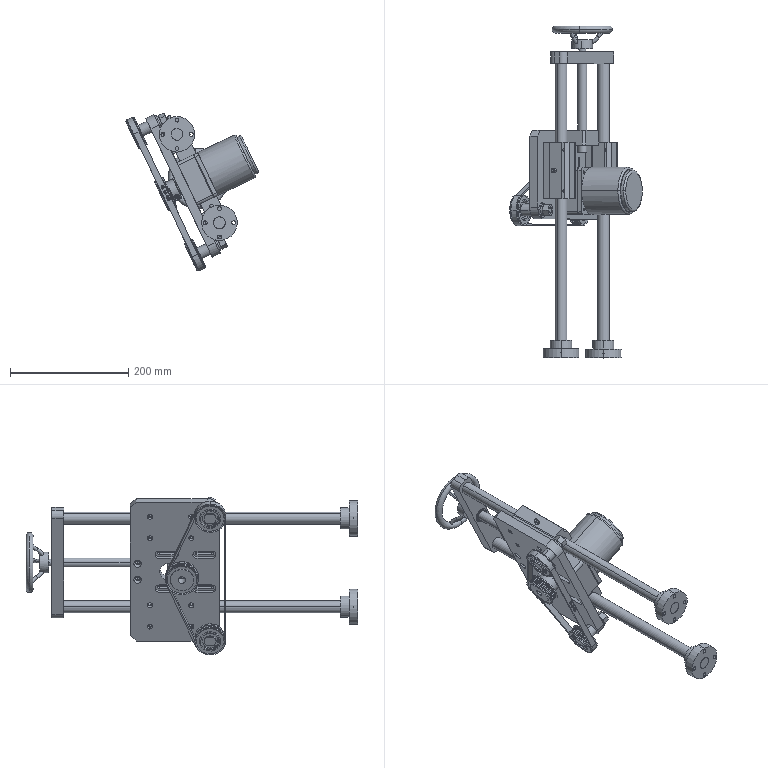Assembly | SolidWorks | mm | 32 component files | 32 solids | 1935 faces | box 224.34 x 561.5 x 267.03 mm | volume 2250519 mm3 | cylinder 1205 | plane 397 | cone 122 | torus 104 | spline 73 | sphere 34 | commonest cylinder face diameters 1.1 x224 0.5 x212 6.55 x196 46.79 x62 43.25 x60 46.43 x33 20 x32 49.97 x32
Bill of materials:
20OpticalAxis1-1 | 2 |  | Long, slender solid cylindrical rod with a constant diameter and plain flat ends.
25WMotor | 1 |  | Motor-like body: a cylindrical housing with a stepped, rounded rear end cap, joined to a square flange and a rectangular front block that has an output shaft sticking out of it.
AHTF30S5M100body | 2 |  | Toothed pulley-like ring: a short cylinder with axial teeth around its outside, a flange at each end, and a large central bore.
bearingB6201ZZ | 2 |  | Short annular ring with flat faces, a central bore, and concentric circular lines on the faces, looking like a simplified bearing.
RTWN32 | 2 |  | Thin, flat, open circular ring of constant thickness, with a lug at each end of the gap and a small hole through each lug, shaped like an internal retaining ring.
Bearing | 2 |  | Rectangular block housing with a large axial through-bore, stepped/chamfered side faces, mounting holes on the top and side faces, and a small fitting on the top, looking like a linear bushing block.
Rolling bearings 61901 GB 276-94 | 1 |  | Annular rolling-element assembly shaped like a radial ball bearing: concentric outer and inner rings with one ring of spherical balls between them, open on the visible face.
DowelPin1-1 | 2 |  | Headed stepped pin: a round head flange, a long cylindrical shank, and a shorter, smaller-diameter end, with a small ring/groove at the step.
FeedingOpticalAxisFrameConnector1-1 | 1 |  | Flat bar link with rounded ends: two small holes near the ends and a larger hole in the middle, with counterbores or chamfers on one face.
FeedingPressingPlate1-1 | 1 |  | Rectangular flat plate with one rounded and one chamfered corner, a central obround slot, four parallel slots, and many through-holes of several sizes in symmetric patterns.
FeedingPressingPlateAdjustmentBlock1-1 | 1 |  | Rectangular block with chamfers on two opposite edges and a single round through-hole crossing it.
FeedingPressingScrew1-1 | 1 |  | Solid stepped cylindrical shaft: a long main diameter that steps down twice to smaller diameters at one end.
Handle1-1 | 1 |  | Handwheel-like part: a toroidal rim joined by three curved spokes to a cylindrical hub that sits off the rim's plane and has a small central bore.
GB_FASTENER_NUT_SNAB1XY M12X1.5-N | 2 |  | Hexagonal prism with a central through-bore, shaped like a hex nut, with chamfered corners on both end faces.
HTCPA32_S5M100_12pulley | 1 |  | Toothed pulley: a cylindrical body with axial teeth around its outside, a flange on each side of the toothed section, and a cylindrical hub on one side. The hub has a central bore and a radial slit, which looks like a clamping hub.
Slotted_head_cap_screw_ISO_4762_M4x16 | 1 |  | Headed fastener: a cylindrical head with a hexagonal socket recess, a plain straight cylindrical shank, and a chamfered tip. The shape matches a socket-head cap screw.
OpticalAxisSeat1-1 | 2 |  | Flanged bushing or flange nut body: a round flange with a smaller cylindrical boss on one side, a central through bore, and four evenly spaced through holes on a bolt circle in the flange.
GB_FASTENER_WASHER_PWNA 12 | 2 |  | Thin, flat, plain annular disc with a central circular hole, shaped like a flat washer.
GB_FASTENER_WASHER_SW 12 | 2 |  | Ring with a rectangular cross-section and one radial split through the ring, shaped like a split (spring) lock washer.
TimingBelt5M-10-625 | 1 |  | Thin closed-loop band of constant width and thickness, shaped like a rounded triangle: one long straight side and two shorter sides meeting at rounded corners.
Washer1-1 | 2 |  | Plain cylindrical tube: a hollow cylinder with a concentric through bore and flat, square-cut ends, shaped like a spacer or sleeve.
Mates:
1. coincident | 20OpticalAxis1-1-1 face at (-30.965, 0, 663.073) dir (0, -1, 0) | assembly plane at (0, 0, 0) dir (0, 1, 0)
2. concentric | 20OpticalAxis1-1-1 face at (-30.965, 0, 663.073) dir (0, 1, 0) r 10 | Bearing-2 face at (-30.965, 269, 663.073) dir (0, -1, 0) r 10
3. concentric | 20OpticalAxis1-1-2 face at (40.711, 0, 513.345) dir (0, 1, 0) r 10 | Bearing-1 face at (40.711, 269, 513.345) dir (0, -1, 0) r 10
4. coincident | 20OpticalAxis1-1-1 face at (-30.965, 0, 663.073) dir (0, -1, 0) | 20OpticalAxis1-1-2 face at (40.711, 0, 513.345) dir (0, -1, 0)
5. coincident | Bearing-1 face at (33.428, 365, 479.924) dir (-0.902, 0, -0.4318) | Bearing-2 face at (-38.248, 365, 629.652) dir (-0.902, 0, -0.4318)
6. coincident | Bearing-1 face at (70.409, 365, 497.627) dir (0, 1, 0) | Bearing-2 face at (-1.267, 365, 647.355) dir (0, 1, 0)
7. concentric | 20OpticalAxis1-1-1 face at (-30.965, 0, 663.073) dir (0, 1, 0) r 10 | OpticalAxisSeat1-1-1 face at (-30.965, -1.22, 663.073) dir (0, -1, 0) r 10
8. coincident | 20OpticalAxis1-1-1 face at (-30.965, 0, 663.073) dir (0, -1, 0) | OpticalAxisSeat1-1-1 face at (-20.965, 0, 663.073) dir (0, -1, 0)
9. concentric | 20OpticalAxis1-1-2 face at (40.711, 0, 513.345) dir (0, 1, 0) r 10 | OpticalAxisSeat1-1-2 face at (40.711, -1.22, 513.345) dir (0, -1, 0) r 10
10. coincident | 20OpticalAxis1-1-2 face at (40.711, 0, 513.345) dir (0, -1, 0) | OpticalAxisSeat1-1-2 face at (50.711, 0, 513.345) dir (0, -1, 0)
11. coincident | Bearing-1 face at (33.428, 365, 479.924) dir (-0.902, 0, -0.4318) | FeedingPressingPlate1-1-1 face at (-70.2, 235, 696.399) dir (0.902, 0, 0.4318)
12. distance | Bearing-1 face at (70.409, 365, 497.627) dir (0, 1, 0) | FeedingPressingPlate1-1-1 face at (-70.2, 385, 696.399) dir (0, 1, 0)
13. distance | Bearing-2 face at (-107.114, 439.5, 656.554) dir (-0.4318, 0, 0.902) | FeedingPressingPlate1-1-1 face at (-70.2, 235, 696.399) dir (-0.4318, 0, 0.902)
14. concentric | FeedingPressingPlate1-1-1 face at (35.587, 250, 475.414) dir (-0.902, 0, -0.4318) r 6 | AHTF30S5M100-1/bearingB6201ZZ-1 face at (-5.002, 250, 455.984) dir (0.902, 0, 0.4318) r 6
15. concentric | FeedingPressingPlate1-1-1 face at (-63.723, 250, 682.869) dir (-0.902, 0, -0.4318) r 6 | AHTF30S5M100-2/bearingB6201ZZ-1 face at (-104.312, 250, 663.439) dir (0.902, 0, 0.4318) r 6
16. coincident | AHTF30S5M100-1/AHTF30S5M100body-1 face at (-10.355, 264.779, 460.218) dir (-0.902, 0, -0.4318) | AHTF30S5M100-2/AHTF30S5M100body-1 face at (-109.665, 264.779, 667.673) dir (-0.902, 0, -0.4318)
17. concentric | AHTF30S5M100-1/bearingB6201ZZ-1 face at (-5.002, 250, 455.984) dir (0.902, 0, 0.4318) r 6 | DowelPin1-1-1 face at (33.783, 250, 474.551) dir (-0.902, 0, -0.4318) r 6
18. coincident | AHTF30S5M100-1/bearingB6201ZZ-1 face at (-6.094, 256.096, 458.265) dir (-0.902, 0, -0.4318) | DowelPin1-1-1 face at (-5.002, 250, 455.984) dir (0.902, 0, 0.4318)
19. concentric | DowelPin1-1-1 face at (33.783, 250, 474.551) dir (-0.902, 0, -0.4318) r 6 | Washer1-1-1 face at (22.057, 250, 468.937) dir (-0.902, 0, -0.4318) r 6.25
20. coincident | AHTF30S5M100-1/bearingB6201ZZ-1 face at (2.578, 258.036, 463.308) dir (0.902, 0, 0.4318) | Washer1-1-1 face at (4.018, 250, 460.302) dir (-0.902, 0, -0.4318)
21. coincident | FeedingPressingPlate1-1-1 face at (-83.73, 235, 689.922) dir (-0.902, 0, -0.4318) | Washer1-1-1 face at (22.057, 250, 468.937) dir (0.902, 0, 0.4318)
22. concentric | DowelPin1-1-1 face at (49.116, 250, 481.891) dir (-0.902, 0, -0.4318) r 5.188 | hex nuts 1-fine pitch-grades ab gb-1 face at (40.638, 250, 477.832) dir (0.902, 0, 0.4318) r 523.599
23. coincident | hex nuts 1-fine pitch-grades ab gb-1 face at (38.394, 241, 482.519) dir (-0.902, 0, -0.4318) | spring lock washers--normal type gb-1 face at (40.638, 250, 477.832) dir (0.902, 0, 0.4318)
24. concentric | DowelPin1-1-1 face at (49.116, 250, 481.891) dir (-0.902, 0, -0.4318) r 5.188 | plain washers-n series-grade a gb-1 face at (37.842, 250, 476.494) dir (-0.902, 0, -0.4318) r 6.5
25. concentric | plain washers-n series-grade a gb-1 face at (37.842, 250, 476.494) dir (-0.902, 0, -0.4318) r 12 | spring lock washers--normal type gb-1 face at (37.842, 250, 476.494) dir (0.902, 0, 0.4318) r 6.45
26. coincident | plain washers-n series-grade a gb-1 face at (37.842, 250, 476.494) dir (0.902, 0, 0.4318) | spring lock washers--normal type gb-1 face at (37.842, 250, 476.494) dir (-0.902, 0, -0.4318)
27. coincident | FeedingPressingPlate1-1-1 face at (-70.2, 235, 696.399) dir (0.902, 0, 0.4318) | plain washers-n series-grade a gb-1 face at (35.587, 250, 475.414) dir (-0.902, 0, -0.4318)
28. concentric | AHTF30S5M100-2/bearingB6201ZZ-1 face at (-104.312, 250, 663.439) dir (0.902, 0, 0.4318) r 6 | DowelPin1-1-2 face at (-65.527, 250, 682.005) dir (-0.902, 0, -0.4318) r 6
29. coincident | AHTF30S5M100-2/bearingB6201ZZ-1 face at (-105.404, 256.096, 665.72) dir (-0.902, 0, -0.4318) | DowelPin1-1-2 face at (-104.312, 250, 663.439) dir (0.902, 0, 0.4318)
30. concentric | DowelPin1-1-2 face at (-65.527, 250, 682.005) dir (-0.902, 0, -0.4318) r 6 | Washer1-1-2 face at (-77.253, 250, 676.392) dir (-0.902, 0, -0.4318) r 10
31. coincident | AHTF30S5M100-2/bearingB6201ZZ-1 face at (-96.732, 258.036, 670.763) dir (0.902, 0, 0.4318) | Washer1-1-2 face at (-95.293, 250, 667.757) dir (-0.902, 0, -0.4318)
32. concentric | DowelPin1-1-2 face at (-50.194, 250, 689.346) dir (-0.902, 0, -0.4318) r 5.188 | hex nuts 1-fine pitch-grades ab gb-2 face at (-58.672, 250, 685.287) dir (0.902, 0, 0.4318) r 523.599
33. coincident | spring lock washers--normal type gb-2 face at (-58.672, 250, 685.287) dir (0.902, 0, 0.4318) | hex nuts 1-fine pitch-grades ab gb-2 face at (-60.916, 241, 689.974) dir (-0.902, 0, -0.4318)
34. concentric | DowelPin1-1-2 face at (-50.194, 250, 689.346) dir (-0.902, 0, -0.4318) r 5.188 | spring lock washers--normal type gb-2 face at (-61.469, 250, 683.948) dir (0.902, 0, 0.4318) r 6.45
35. concentric | DowelPin1-1-2 face at (-50.194, 250, 689.346) dir (-0.902, 0, -0.4318) r 5.188 | plain washers-n series-grade a gb-2 face at (-61.469, 250, 683.948) dir (-0.902, 0, -0.4318) r 6.5
36. coincident | FeedingPressingPlate1-1-1 face at (-70.2, 235, 696.399) dir (0.902, 0, 0.4318) | plain washers-n series-grade a gb-2 face at (-63.723, 250, 682.869) dir (-0.902, 0, -0.4318)
37. coincident | spring lock washers--normal type gb-2 face at (-61.469, 250, 683.948) dir (-0.902, 0, -0.4318) | plain washers-n series-grade a gb-2 face at (-61.469, 250, 683.948) dir (0.902, 0, 0.4318)
38. coincident | AHTF30S5M100-2/AHTF30S5M100body-1 face at (-108.713, 272.053, 671.474) dir (0.902, 0, 0.4318) | HTCPA32_S5M100_12-1/HTCPA32_S5M100_12pulley-1 face at (-55.827, 272.581, 560.996) dir (0.902, 0, 0.4318)
39. coincident | FeedingPressingPlate1-1-1 face at (-70.2, 235, 696.399) dir (0.902, 0, 0.4318) | 25WMotor-1 face at (-14.068, 282.511, 579.142) dir (-0.902, 0, -0.4318)
40. distance | TimingBelt5M-10-625-1 face at (-104.312, 250, 663.439) dir (-0.902, 0, -0.4318) | AHTF30S5M100-2/AHTF30S5M100body-1 face at (-108.713, 272.053, 671.474) dir (0.902, 0, 0.4318)
41. concentric | AHTF30S5M100-2/AHTF30S5M100body-1 edge at (-94.842, 250, 667.972) dir (0.902, 0, 0.4318) r 23.875 | TimingBelt5M-10-625-1 face at (-95.293, 250, 667.757) dir (-0.902, 0, -0.4318) r 26.55
42. concentric | AHTF30S5M100-1/AHTF30S5M100body-1 edge at (4.469, 250, 460.518) dir (0.902, 0, 0.4318) r 23.875 | TimingBelt5M-10-625-1 face at (4.018, 250, 460.302) dir (-0.902, 0, -0.4318) r 26.55
43. distance | FeedingPressingPlate1-1-1 face at (-70.2, 385, 696.399) dir (0, 1, 0) | 20OpticalAxis1-1-2 face at (40.711, 500, 513.345) dir (0, 1, 0)
44. concentric | 20OpticalAxis1-1-2 face at (40.711, 0, 513.345) dir (0, 1, 0) r 10 | FeedingOpticalAxisFrameConnector1-1-1 face at (40.711, 518, 513.345) dir (0, 1, 0) r 4.5
45. coincident | FeedingPressingPlate1-1-1 face at (-70.2, 235, 696.399) dir (0.902, 0, 0.4318) | FeedingPressingPlateAdjustmentBlock1-1-1 face at (-27.022, 360, 606.201) dir (-0.902, 0, -0.4318)
46. coincident | FeedingPressingPlate1-1-1 face at (-70.2, 385, 696.399) dir (0, 1, 0) | FeedingPressingPlateAdjustmentBlock1-1-1 face at (9.057, 385, 623.472) dir (0, 1, 0)
47. width | FeedingPressingPlateAdjustmentBlock1-1-1 face at (34.964, 360, 569.354) dir (0.4318, 0, -0.902) | FeedingPressingPlateAdjustmentBlock1-1-1 face at (9.057, 360, 623.472) dir (-0.4318, 0, 0.902) | FeedingPressingPlate1-1-1 face at (-70.2, 235, 696.399) dir (-0.4318, 0, 0.902) | FeedingPressingPlate1-1-1 face at (42.063, 235, 461.884) dir (0.4318, 0, -0.902)
48. concentric | FeedingOpticalAxisFrameConnector1-1-1 face at (4.873, 518, 588.209) dir (0, 1, 0) r 9 | FeedingPressingScrew1-1-1 face at (4.873, 513, 588.209) dir (0, -1, 0) r 6
49. coincident | FeedingOpticalAxisFrameConnector1-1-1 face at (-51.835, 498, 671.93) dir (0, -1, 0) | FeedingPressingScrew1-1-1 face at (4.873, 498, 588.209) dir (0, 1, 0)
50. concentric | FeedingPressingScrew1-1-1 face at (4.873, 533, 588.209) dir (0, -1, 0) r 4 | Handle1-1-1 face at (4.873, 523, 588.209) dir (0, 1, 0) r 4
51. coincident | FeedingPressingScrew1-1-1 face at (4.873, 523, 588.209) dir (0, 1, 0) | Handle1-1-1 face at (4.873, 523, 588.209) dir (0, -1, 0)
52. concentric | 20OpticalAxis1-1-1 face at (-30.965, 0, 663.073) dir (0, 1, 0) r 10 | FeedingOpticalAxisFrameConnector1-1-1 face at (-30.965, 500, 663.073) dir (0, -1, 0) r 10
53. coincident | 20OpticalAxis1-1-1 face at (-30.965, 500, 663.073) dir (0, 1, 0) | FeedingOpticalAxisFrameConnector1-1-1 face at (-30.965, 500, 663.073) dir (0, -1, 0)
54. slot | 25WMotor-1 face at (-0.3291, 250.691, 550.441) dir (-0.902, 0, -0.4318) r 2.1 | FeedingPressingPlate1-1-1 face at (-1.732, 247.329, 553.372) dir (0.4318, 0, -0.902)
55. slot | 25WMotor-1 face at (-0.3291, 314.33, 550.441) dir (-0.902, 0, -0.4318) r 2.1 | FeedingPressingPlate1-1-1 face at (-1.732, 335.968, 553.372) dir (0.4318, 0, -0.902)
56. concentric | HTCPA32_S5M100_12-1/HTCPA32_S5M100_12pulley-1 face at (-30.304, 297.511, 571.369) dir (-0.902, 0, -0.4318) r 6 | 25WMotor-1 face at (-42.932, 297.511, 565.324) dir (0.902, 0, 0.4318) r 5
57. concentric | FeedingPressingScrew1-1-1 face at (4.873, 523, 588.209) dir (0, -1, 0) r 5.9 | deep groove ball bearings gb-1 face at (4.873, 494.029, 588.209) dir (0, -1, 0) r 6
58. coincident | FeedingOpticalAxisFrameConnector1-1-1 face at (4.873, 504, 588.209) dir (0, -1, 0) | deep groove ball bearings gb-1 face at (8.106, 504, 599.765) dir (0, 1, 0)
59. coincident | AHTF30S5M100body-1 plane at (3, 0, 0) dir (1, 0, 0) | bearingB6201ZZ-1 plane at (3, 0, 0) dir (1, 0, 0)
60. coincident | AHTF30S5M100body-1 axis at (80.9, 0, 0) dir (-1, 0, 0) | bearingB6201ZZ-1 axis at (83.9, 0, 0) dir (-1, 0, 0)
61. coincident | AHTF30S5M100body-1 plane at (13, 0, 0) dir (1, 0, 0) | RTWN32-1 plane at (13, 0, 0) dir (1, 0, 0)
62. coincident | AHTF30S5M100body-1 axis at (80.9, 0, 0) dir (-1, 0, 0) | RTWN32-1 axis at (94.5, 0, 0) dir (-1, 0, 0)
63. coincident | HTCPA32_S5M100_12pulley-1 axis at (23.7, 50, 13.2) dir (0, -1, 0) | Slotted_head_cap_screw_ISO_4762_M4x16-1 axis at (23.7, -75.5, 13.2) dir (0, 1, 0)